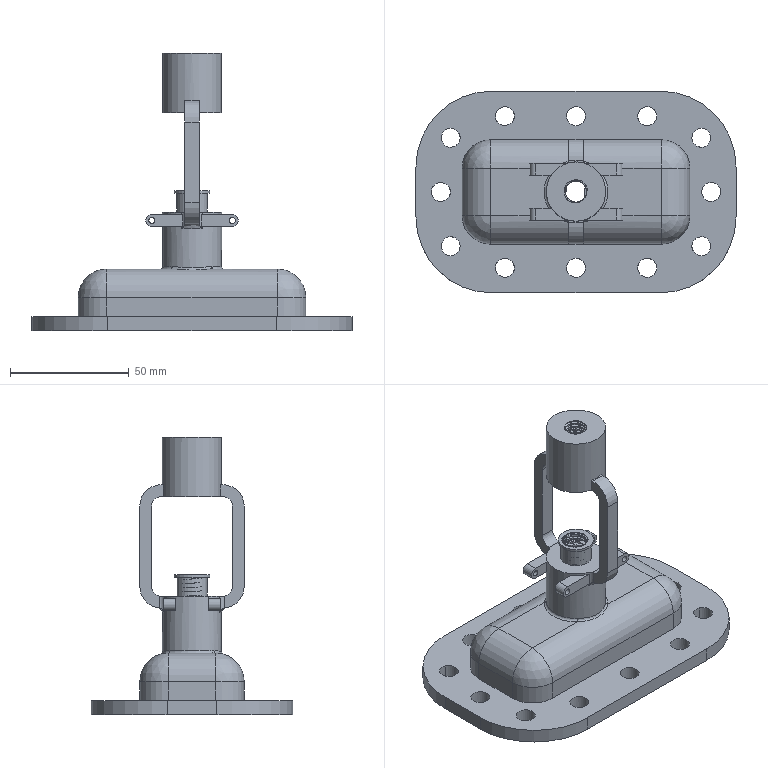Component | NX | TOP_COVER | 1 solid | 154 faces | volume 85958 mm3 | cylinder 86 | plane 50 | sphere 8 | spline 8 | torus 2 | commonest cylinder face diameters 10.2 x22 8 x20 18 x12 24 x8 4 x4 64 x4 5 x4 2.5 x4